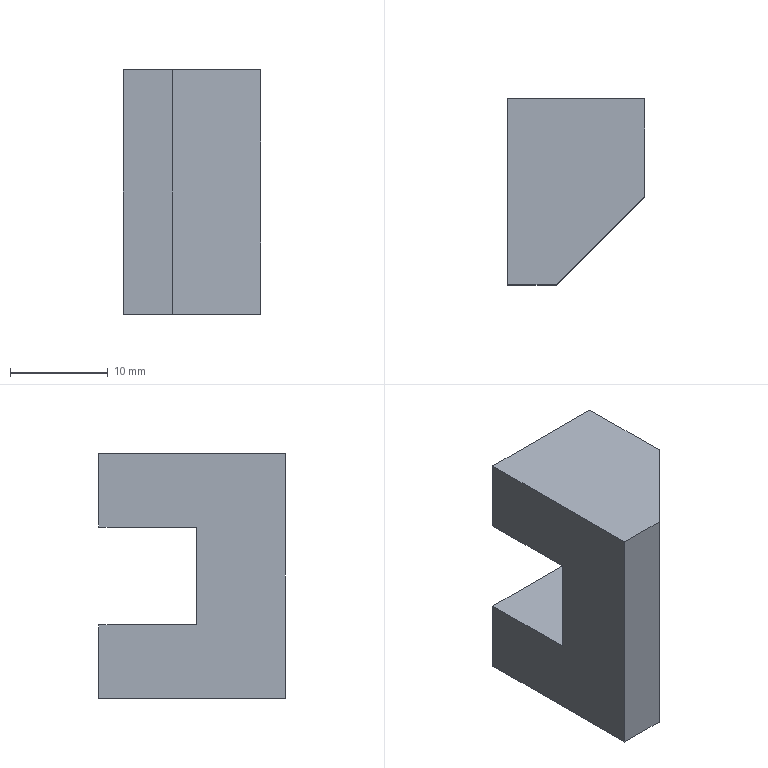Component | NX | CON_ROD4 | 1 solid | 12 faces | box 14 x 19 x 25 mm | volume 4238 mm3 | plane 12
STEP:
#1=CARTESIAN_POINT('',(0.,0.,0.));
#2=DIRECTION('',(0.,0.,1.));
#3=DIRECTION('',(1.,0.,0.));
#4=AXIS2_PLACEMENT_3D('',#1,#2,#3);
#5=CARTESIAN_POINT('',(101.5,69.,38.5));
#6=VERTEX_POINT('',#5);
#7=CARTESIAN_POINT('',(101.5,59.,38.5));
#8=VERTEX_POINT('',#7);
#9=CARTESIAN_POINT('',(101.5,69.,38.5));
#10=DIRECTION('',(0.,-1.,-0.));
#11=VECTOR('',#10,1.);
#12=LINE('',#9,#11);
#13=CARTESIAN_POINT('',(101.5,69.,26.));
#14=DIRECTION('',(1.,0.,0.));
#15=DIRECTION('',(0.,1.,0.));
#16=AXIS2_PLACEMENT_3D('',#13,#14,#15);
#17=PLANE('',#16);
#18=CARTESIAN_POINT('',(0.,12.5));
#19=DIRECTION('',(-1.,-0.));
#20=VECTOR('',#19,1.);
#21=LINE('',#18,#20);
#22=(GEOMETRIC_REPRESENTATION_CONTEXT(2)PARAMETRIC_REPRESENTATION_CONTEXT()REPRESENTATION_CONTEXT('',''));
#23=DEFINITIONAL_REPRESENTATION('',(#21),#22);
#24=PCURVE('',#17,#23);
#25=CARTESIAN_POINT('',(101.5,69.,38.5));
#26=DIRECTION('',(0.,0.,-1.));
#27=DIRECTION('',(0.,1.,0.));
#28=AXIS2_PLACEMENT_3D('',#25,#26,#27);
#29=PLANE('',#28);
#30=CARTESIAN_POINT('',(0.,0.));
#31=DIRECTION('',(-1.,0.));
#32=VECTOR('',#31,1.);
#33=LINE('',#30,#32);
#34=(GEOMETRIC_REPRESENTATION_CONTEXT(2)PARAMETRIC_REPRESENTATION_CONTEXT()REPRESENTATION_CONTEXT('',''));
#35=DEFINITIONAL_REPRESENTATION('',(#33),#34);
#36=PCURVE('',#29,#35);
#37=SURFACE_CURVE('',#12,(#24,#36),.PCURVE_S1.);
#38=EDGE_CURVE('',#6,#8,#37,.T.);
#39=ORIENTED_EDGE('',*,*,#38,.T.);
#40=CARTESIAN_POINT('',(101.5,59.,31.));
#41=VERTEX_POINT('',#40);
#42=CARTESIAN_POINT('',(101.5,59.,13.5));
#43=DIRECTION('',(0.,0.,-1.));
#44=VECTOR('',#43,1.);
#45=LINE('',#42,#44);
#46=CARTESIAN_POINT('',(-10.,-12.5));
#47=DIRECTION('',(0.,-1.));
#48=VECTOR('',#47,1.);
#49=LINE('',#46,#48);
#50=(GEOMETRIC_REPRESENTATION_CONTEXT(2)PARAMETRIC_REPRESENTATION_CONTEXT()REPRESENTATION_CONTEXT('',''));
#51=DEFINITIONAL_REPRESENTATION('',(#49),#50);
#52=PCURVE('',#17,#51);
#53=CARTESIAN_POINT('',(101.5,59.,26.));
#54=DIRECTION('',(0.7071,-0.7071,0.));
#55=DIRECTION('',(0.,0.,1.));
#56=AXIS2_PLACEMENT_3D('',#53,#54,#55);
#57=PLANE('',#56);
#58=CARTESIAN_POINT('',(-12.5,0.));
#59=DIRECTION('',(-1.,0.));
#60=VECTOR('',#59,1.);
#61=LINE('',#58,#60);
#62=(GEOMETRIC_REPRESENTATION_CONTEXT(2)PARAMETRIC_REPRESENTATION_CONTEXT()REPRESENTATION_CONTEXT('',''));
#63=DEFINITIONAL_REPRESENTATION('',(#61),#62);
#64=PCURVE('',#57,#63);
#65=SURFACE_CURVE('',#45,(#52,#64),.PCURVE_S1.);
#66=EDGE_CURVE('',#8,#41,#65,.T.);
#67=ORIENTED_EDGE('',*,*,#66,.T.);
#68=CARTESIAN_POINT('',(101.5,69.,31.));
#69=VERTEX_POINT('',#68);
#70=CARTESIAN_POINT('',(101.5,59.,31.));
#71=DIRECTION('',(0.,1.,0.));
#72=VECTOR('',#71,1.);
#73=LINE('',#70,#72);
#74=CARTESIAN_POINT('',(-10.,5.));
#75=DIRECTION('',(1.,0.));
#76=VECTOR('',#75,1.);
#77=LINE('',#74,#76);
#78=(GEOMETRIC_REPRESENTATION_CONTEXT(2)PARAMETRIC_REPRESENTATION_CONTEXT()REPRESENTATION_CONTEXT('',''));
#79=DEFINITIONAL_REPRESENTATION('',(#77),#78);
#80=PCURVE('',#17,#79);
#81=CARTESIAN_POINT('',(101.5,59.,31.));
#82=DIRECTION('',(0.,-0.,1.));
#83=DIRECTION('',(0.,-1.,-0.));
#84=AXIS2_PLACEMENT_3D('',#81,#82,#83);
#85=PLANE('',#84);
#86=CARTESIAN_POINT('',(0.,0.));
#87=DIRECTION('',(-1.,0.));
#88=VECTOR('',#87,1.);
#89=LINE('',#86,#88);
#90=(GEOMETRIC_REPRESENTATION_CONTEXT(2)PARAMETRIC_REPRESENTATION_CONTEXT()REPRESENTATION_CONTEXT('',''));
#91=DEFINITIONAL_REPRESENTATION('',(#89),#90);
#92=PCURVE('',#85,#91);
#93=SURFACE_CURVE('',#73,(#80,#92),.PCURVE_S1.);
#94=EDGE_CURVE('',#41,#69,#93,.T.);
#95=ORIENTED_EDGE('',*,*,#94,.T.);
#96=CARTESIAN_POINT('',(101.5,69.,31.));
#97=DIRECTION('',(0.,0.,1.));
#98=VECTOR('',#97,1.);
#99=LINE('',#96,#98);
#100=CARTESIAN_POINT('',(0.,5.));
#101=DIRECTION('',(0.,1.));
#102=VECTOR('',#101,1.);
#103=LINE('',#100,#102);
#104=(GEOMETRIC_REPRESENTATION_CONTEXT(2)PARAMETRIC_REPRESENTATION_CONTEXT()REPRESENTATION_CONTEXT('',''));
#105=DEFINITIONAL_REPRESENTATION('',(#103),#104);
#106=PCURVE('',#17,#105);
#107=CARTESIAN_POINT('',(101.5,69.,31.));
#108=DIRECTION('',(0.,-1.,0.));
#109=DIRECTION('',(1.,0.,0.));
#110=AXIS2_PLACEMENT_3D('',#107,#108,#109);
#111=PLANE('',#110);
#112=CARTESIAN_POINT('',(0.,0.));
#113=DIRECTION('',(0.,1.));
#114=VECTOR('',#113,1.);
#115=LINE('',#112,#114);
#116=(GEOMETRIC_REPRESENTATION_CONTEXT(2)PARAMETRIC_REPRESENTATION_CONTEXT()REPRESENTATION_CONTEXT('',''));
#117=DEFINITIONAL_REPRESENTATION('',(#115),#116);
#118=PCURVE('',#111,#117);
#119=SURFACE_CURVE('',#99,(#106,#118),.PCURVE_S1.);
#120=EDGE_CURVE('',#69,#6,#119,.T.);
#121=ORIENTED_EDGE('',*,*,#120,.T.);
#122=EDGE_LOOP('',(#39,#67,#95,#121));
#123=FACE_BOUND('',#122,.T.);
#124=ADVANCED_FACE('',(#123),#17,.T.);
#125=CARTESIAN_POINT('',(101.5,59.,13.5));
#126=VERTEX_POINT('',#125);
#127=CARTESIAN_POINT('',(101.5,69.,13.5));
#128=VERTEX_POINT('',#127);
#129=CARTESIAN_POINT('',(101.5,50.,13.5));
#130=DIRECTION('',(0.,1.,0.));
#131=VECTOR('',#130,1.);
#132=LINE('',#129,#131);
#133=CARTESIAN_POINT('',(101.5,50.,13.5));
#134=DIRECTION('',(0.,-0.,1.));
#135=DIRECTION('',(0.,-1.,-0.));
#136=AXIS2_PLACEMENT_3D('',#133,#134,#135);
#137=PLANE('',#136);
#138=CARTESIAN_POINT('',(0.,0.));
#139=DIRECTION('',(-1.,0.));
#140=VECTOR('',#139,1.);
#141=LINE('',#138,#140);
#142=(GEOMETRIC_REPRESENTATION_CONTEXT(2)PARAMETRIC_REPRESENTATION_CONTEXT()REPRESENTATION_CONTEXT('',''));
#143=DEFINITIONAL_REPRESENTATION('',(#141),#142);
#144=PCURVE('',#137,#143);
#145=CARTESIAN_POINT('',(101.5,69.,26.));
#146=DIRECTION('',(1.,0.,0.));
#147=DIRECTION('',(0.,1.,0.));
#148=AXIS2_PLACEMENT_3D('',#145,#146,#147);
#149=PLANE('',#148);
#150=CARTESIAN_POINT('',(-19.,-12.5));
#151=DIRECTION('',(1.,0.));
#152=VECTOR('',#151,1.);
#153=LINE('',#150,#152);
#154=(GEOMETRIC_REPRESENTATION_CONTEXT(2)PARAMETRIC_REPRESENTATION_CONTEXT()REPRESENTATION_CONTEXT('',''));
#155=DEFINITIONAL_REPRESENTATION('',(#153),#154);
#156=PCURVE('',#149,#155);
#157=SURFACE_CURVE('',#132,(#144,#156),.PCURVE_S1.);
#158=EDGE_CURVE('',#126,#128,#157,.T.);
#159=ORIENTED_EDGE('',*,*,#158,.F.);
#160=CARTESIAN_POINT('',(92.5,50.,13.5));
#161=VERTEX_POINT('',#160);
#162=CARTESIAN_POINT('',(101.5,59.,13.5));
#163=DIRECTION('',(-0.7071,-0.7071,-0.));
#164=VECTOR('',#163,1.);
#165=LINE('',#162,#164);
#166=CARTESIAN_POINT('',(-9.,0.));
#167=DIRECTION('',(0.7071,-0.7071));
#168=VECTOR('',#167,1.);
#169=LINE('',#166,#168);
#170=(GEOMETRIC_REPRESENTATION_CONTEXT(2)PARAMETRIC_REPRESENTATION_CONTEXT()REPRESENTATION_CONTEXT('',''));
#171=DEFINITIONAL_REPRESENTATION('',(#169),#170);
#172=PCURVE('',#137,#171);
#173=CARTESIAN_POINT('',(-12.5,0.));
#174=DIRECTION('',(-0.,1.));
#175=VECTOR('',#174,1.);
#176=LINE('',#173,#175);
#177=(GEOMETRIC_REPRESENTATION_CONTEXT(2)PARAMETRIC_REPRESENTATION_CONTEXT()REPRESENTATION_CONTEXT('',''));
#178=DEFINITIONAL_REPRESENTATION('',(#176),#177);
#179=PCURVE('',#57,#178);
#180=SURFACE_CURVE('',#165,(#172,#179),.PCURVE_S1.);
#181=EDGE_CURVE('',#126,#161,#180,.T.);
#182=ORIENTED_EDGE('',*,*,#181,.T.);
#183=CARTESIAN_POINT('',(87.5,50.,13.5));
#184=VERTEX_POINT('',#183);
#185=CARTESIAN_POINT('',(101.5,50.,13.5));
#186=DIRECTION('',(-1.,0.,0.));
#187=VECTOR('',#186,1.);
#188=LINE('',#185,#187);
#189=CARTESIAN_POINT('',(0.,0.));
#190=DIRECTION('',(0.,-1.));
#191=VECTOR('',#190,1.);
#192=LINE('',#189,#191);
#193=(GEOMETRIC_REPRESENTATION_CONTEXT(2)PARAMETRIC_REPRESENTATION_CONTEXT()REPRESENTATION_CONTEXT('',''));
#194=DEFINITIONAL_REPRESENTATION('',(#192),#193);
#195=PCURVE('',#137,#194);
#196=CARTESIAN_POINT('',(101.5,50.,38.5));
#197=DIRECTION('',(0.,1.,0.));
#198=DIRECTION('',(-1.,0.,0.));
#199=AXIS2_PLACEMENT_3D('',#196,#197,#198);
#200=PLANE('',#199);
#201=CARTESIAN_POINT('',(0.,-25.));
#202=DIRECTION('',(1.,0.));
#203=VECTOR('',#202,1.);
#204=LINE('',#201,#203);
#205=(GEOMETRIC_REPRESENTATION_CONTEXT(2)PARAMETRIC_REPRESENTATION_CONTEXT()REPRESENTATION_CONTEXT('',''));
#206=DEFINITIONAL_REPRESENTATION('',(#204),#205);
#207=PCURVE('',#200,#206);
#208=SURFACE_CURVE('',#188,(#195,#207),.PCURVE_S1.);
#209=EDGE_CURVE('',#161,#184,#208,.T.);
#210=ORIENTED_EDGE('',*,*,#209,.T.);
#211=CARTESIAN_POINT('',(87.5,69.,13.5));
#212=VERTEX_POINT('',#211);
#213=CARTESIAN_POINT('',(87.5,50.,13.5));
#214=DIRECTION('',(0.,1.,0.));
#215=VECTOR('',#214,1.);
#216=LINE('',#213,#215);
#217=CARTESIAN_POINT('',(0.,-14.));
#218=DIRECTION('',(-1.,0.));
#219=VECTOR('',#218,1.);
#220=LINE('',#217,#219);
#221=(GEOMETRIC_REPRESENTATION_CONTEXT(2)PARAMETRIC_REPRESENTATION_CONTEXT()REPRESENTATION_CONTEXT('',''));
#222=DEFINITIONAL_REPRESENTATION('',(#220),#221);
#223=PCURVE('',#137,#222);
#224=CARTESIAN_POINT('',(87.5,69.,26.));
#225=DIRECTION('',(1.,0.,0.));
#226=DIRECTION('',(0.,1.,0.));
#227=AXIS2_PLACEMENT_3D('',#224,#225,#226);
#228=PLANE('',#227);
#229=CARTESIAN_POINT('',(-19.,-12.5));
#230=DIRECTION('',(1.,0.));
#231=VECTOR('',#230,1.);
#232=LINE('',#229,#231);
#233=(GEOMETRIC_REPRESENTATION_CONTEXT(2)PARAMETRIC_REPRESENTATION_CONTEXT()REPRESENTATION_CONTEXT('',''));
#234=DEFINITIONAL_REPRESENTATION('',(#232),#233);
#235=PCURVE('',#228,#234);
#236=SURFACE_CURVE('',#216,(#223,#235),.PCURVE_S1.);
#237=EDGE_CURVE('',#184,#212,#236,.T.);
#238=ORIENTED_EDGE('',*,*,#237,.T.);
#239=CARTESIAN_POINT('',(101.5,69.,13.5));
#240=DIRECTION('',(-1.,0.,0.));
#241=VECTOR('',#240,1.);
#242=LINE('',#239,#241);
#243=CARTESIAN_POINT('',(-19.,0.));
#244=DIRECTION('',(0.,-1.));
#245=VECTOR('',#244,1.);
#246=LINE('',#243,#245);
#247=(GEOMETRIC_REPRESENTATION_CONTEXT(2)PARAMETRIC_REPRESENTATION_CONTEXT()REPRESENTATION_CONTEXT('',''));
#248=DEFINITIONAL_REPRESENTATION('',(#246),#247);
#249=PCURVE('',#137,#248);
#250=CARTESIAN_POINT('',(101.5,69.,13.5));
#251=DIRECTION('',(0.,-1.,0.));
#252=DIRECTION('',(1.,0.,0.));
#253=AXIS2_PLACEMENT_3D('',#250,#251,#252);
#254=PLANE('',#253);
#255=CARTESIAN_POINT('',(0.,0.));
#256=DIRECTION('',(-1.,0.));
#257=VECTOR('',#256,1.);
#258=LINE('',#255,#257);
#259=(GEOMETRIC_REPRESENTATION_CONTEXT(2)PARAMETRIC_REPRESENTATION_CONTEXT()REPRESENTATION_CONTEXT('',''));
#260=DEFINITIONAL_REPRESENTATION('',(#258),#259);
#261=PCURVE('',#254,#260);
#262=SURFACE_CURVE('',#242,(#249,#261),.PCURVE_S1.);
#263=EDGE_CURVE('',#128,#212,#262,.T.);
#264=ORIENTED_EDGE('',*,*,#263,.F.);
#265=EDGE_LOOP('',(#159,#182,#210,#238,#264));
#266=FACE_BOUND('',#265,.T.);
#267=ADVANCED_FACE('',(#266),#137,.F.);
#268=CARTESIAN_POINT('',(87.5,69.,21.));
#269=VERTEX_POINT('',#268);
#270=CARTESIAN_POINT('',(87.5,69.,13.5));
#271=DIRECTION('',(0.,0.,1.));
#272=VECTOR('',#271,1.);
#273=LINE('',#270,#272);
#274=CARTESIAN_POINT('',(-14.,0.));
#275=DIRECTION('',(0.,1.));
#276=VECTOR('',#275,1.);
#277=LINE('',#274,#276);
#278=(GEOMETRIC_REPRESENTATION_CONTEXT(2)PARAMETRIC_REPRESENTATION_CONTEXT()REPRESENTATION_CONTEXT('',''));
#279=DEFINITIONAL_REPRESENTATION('',(#277),#278);
#280=PCURVE('',#254,#279);
#281=CARTESIAN_POINT('',(0.,-12.5));
#282=DIRECTION('',(0.,1.));
#283=VECTOR('',#282,1.);
#284=LINE('',#281,#283);
#285=(GEOMETRIC_REPRESENTATION_CONTEXT(2)PARAMETRIC_REPRESENTATION_CONTEXT()REPRESENTATION_CONTEXT('',''));
#286=DEFINITIONAL_REPRESENTATION('',(#284),#285);
#287=PCURVE('',#228,#286);
#288=SURFACE_CURVE('',#273,(#280,#287),.PCURVE_S1.);
#289=EDGE_CURVE('',#212,#269,#288,.T.);
#290=ORIENTED_EDGE('',*,*,#289,.T.);
#291=CARTESIAN_POINT('',(101.5,69.,21.));
#292=VERTEX_POINT('',#291);
#293=CARTESIAN_POINT('',(101.5,69.,21.));
#294=DIRECTION('',(-1.,0.,0.));
#295=VECTOR('',#294,1.);
#296=LINE('',#293,#295);
#297=CARTESIAN_POINT('',(0.,7.5));
#298=DIRECTION('',(-1.,0.));
#299=VECTOR('',#298,1.);
#300=LINE('',#297,#299);
#301=(GEOMETRIC_REPRESENTATION_CONTEXT(2)PARAMETRIC_REPRESENTATION_CONTEXT()REPRESENTATION_CONTEXT('',''));
#302=DEFINITIONAL_REPRESENTATION('',(#300),#301);
#303=PCURVE('',#254,#302);
#304=CARTESIAN_POINT('',(101.5,69.,21.));
#305=DIRECTION('',(0.,0.,-1.));
#306=DIRECTION('',(0.,1.,0.));
#307=AXIS2_PLACEMENT_3D('',#304,#305,#306);
#308=PLANE('',#307);
#309=CARTESIAN_POINT('',(0.,0.));
#310=DIRECTION('',(0.,-1.));
#311=VECTOR('',#310,1.);
#312=LINE('',#309,#311);
#313=(GEOMETRIC_REPRESENTATION_CONTEXT(2)PARAMETRIC_REPRESENTATION_CONTEXT()REPRESENTATION_CONTEXT('',''));
#314=DEFINITIONAL_REPRESENTATION('',(#312),#313);
#315=PCURVE('',#308,#314);
#316=SURFACE_CURVE('',#296,(#303,#315),.PCURVE_S1.);
#317=EDGE_CURVE('',#292,#269,#316,.T.);
#318=ORIENTED_EDGE('',*,*,#317,.F.);
#319=CARTESIAN_POINT('',(101.5,69.,13.5));
#320=DIRECTION('',(0.,0.,1.));
#321=VECTOR('',#320,1.);
#322=LINE('',#319,#321);
#323=CARTESIAN_POINT('',(0.,0.));
#324=DIRECTION('',(0.,1.));
#325=VECTOR('',#324,1.);
#326=LINE('',#323,#325);
#327=(GEOMETRIC_REPRESENTATION_CONTEXT(2)PARAMETRIC_REPRESENTATION_CONTEXT()REPRESENTATION_CONTEXT('',''));
#328=DEFINITIONAL_REPRESENTATION('',(#326),#327);
#329=PCURVE('',#254,#328);
#330=CARTESIAN_POINT('',(0.,-12.5));
#331=DIRECTION('',(0.,1.));
#332=VECTOR('',#331,1.);
#333=LINE('',#330,#332);
#334=(GEOMETRIC_REPRESENTATION_CONTEXT(2)PARAMETRIC_REPRESENTATION_CONTEXT()REPRESENTATION_CONTEXT('',''));
#335=DEFINITIONAL_REPRESENTATION('',(#333),#334);
#336=PCURVE('',#149,#335);
#337=SURFACE_CURVE('',#322,(#329,#336),.PCURVE_S1.);
#338=EDGE_CURVE('',#128,#292,#337,.T.);
#339=ORIENTED_EDGE('',*,*,#338,.F.);
#340=ORIENTED_EDGE('',*,*,#263,.T.);
#341=EDGE_LOOP('',(#290,#318,#339,#340));
#342=FACE_BOUND('',#341,.T.);
#343=ADVANCED_FACE('',(#342),#254,.F.);
#344=CARTESIAN_POINT('',(87.5,59.,21.));
#345=VERTEX_POINT('',#344);
#346=CARTESIAN_POINT('',(87.5,69.,21.));
#347=DIRECTION('',(0.,-1.,0.));
#348=VECTOR('',#347,1.);
#349=LINE('',#346,#348);
#350=CARTESIAN_POINT('',(0.,-14.));
#351=DIRECTION('',(-1.,0.));
#352=VECTOR('',#351,1.);
#353=LINE('',#350,#352);
#354=(GEOMETRIC_REPRESENTATION_CONTEXT(2)PARAMETRIC_REPRESENTATION_CONTEXT()REPRESENTATION_CONTEXT('',''));
#355=DEFINITIONAL_REPRESENTATION('',(#353),#354);
#356=PCURVE('',#308,#355);
#357=CARTESIAN_POINT('',(0.,-5.));
#358=DIRECTION('',(-1.,0.));
#359=VECTOR('',#358,1.);
#360=LINE('',#357,#359);
#361=(GEOMETRIC_REPRESENTATION_CONTEXT(2)PARAMETRIC_REPRESENTATION_CONTEXT()REPRESENTATION_CONTEXT('',''));
#362=DEFINITIONAL_REPRESENTATION('',(#360),#361);
#363=PCURVE('',#228,#362);
#364=SURFACE_CURVE('',#349,(#356,#363),.PCURVE_S1.);
#365=EDGE_CURVE('',#269,#345,#364,.T.);
#366=ORIENTED_EDGE('',*,*,#365,.T.);
#367=CARTESIAN_POINT('',(101.5,59.,21.));
#368=VERTEX_POINT('',#367);
#369=CARTESIAN_POINT('',(101.5,59.,21.));
#370=DIRECTION('',(-1.,0.,0.));
#371=VECTOR('',#370,1.);
#372=LINE('',#369,#371);
#373=CARTESIAN_POINT('',(-10.,0.));
#374=DIRECTION('',(0.,-1.));
#375=VECTOR('',#374,1.);
#376=LINE('',#373,#375);
#377=(GEOMETRIC_REPRESENTATION_CONTEXT(2)PARAMETRIC_REPRESENTATION_CONTEXT()REPRESENTATION_CONTEXT('',''));
#378=DEFINITIONAL_REPRESENTATION('',(#376),#377);
#379=PCURVE('',#308,#378);
#380=CARTESIAN_POINT('',(101.5,59.,21.));
#381=DIRECTION('',(0.,-1.,-0.));
#382=DIRECTION('',(0.,0.,-1.));
#383=AXIS2_PLACEMENT_3D('',#380,#381,#382);
#384=PLANE('',#383);
#385=CARTESIAN_POINT('',(0.,0.));
#386=DIRECTION('',(0.,-1.));
#387=VECTOR('',#386,1.);
#388=LINE('',#385,#387);
#389=(GEOMETRIC_REPRESENTATION_CONTEXT(2)PARAMETRIC_REPRESENTATION_CONTEXT()REPRESENTATION_CONTEXT('',''));
#390=DEFINITIONAL_REPRESENTATION('',(#388),#389);
#391=PCURVE('',#384,#390);
#392=SURFACE_CURVE('',#372,(#379,#391),.PCURVE_S1.);
#393=EDGE_CURVE('',#368,#345,#392,.T.);
#394=ORIENTED_EDGE('',*,*,#393,.F.);
#395=CARTESIAN_POINT('',(101.5,69.,21.));
#396=DIRECTION('',(0.,-1.,0.));
#397=VECTOR('',#396,1.);
#398=LINE('',#395,#397);
#399=CARTESIAN_POINT('',(0.,0.));
#400=DIRECTION('',(-1.,0.));
#401=VECTOR('',#400,1.);
#402=LINE('',#399,#401);
#403=(GEOMETRIC_REPRESENTATION_CONTEXT(2)PARAMETRIC_REPRESENTATION_CONTEXT()REPRESENTATION_CONTEXT('',''));
#404=DEFINITIONAL_REPRESENTATION('',(#402),#403);
#405=PCURVE('',#308,#404);
#406=CARTESIAN_POINT('',(0.,-5.));
#407=DIRECTION('',(-1.,0.));
#408=VECTOR('',#407,1.);
#409=LINE('',#406,#408);
#410=(GEOMETRIC_REPRESENTATION_CONTEXT(2)PARAMETRIC_REPRESENTATION_CONTEXT()REPRESENTATION_CONTEXT('',''));
#411=DEFINITIONAL_REPRESENTATION('',(#409),#410);
#412=PCURVE('',#149,#411);
#413=SURFACE_CURVE('',#398,(#405,#412),.PCURVE_S1.);
#414=EDGE_CURVE('',#292,#368,#413,.T.);
#415=ORIENTED_EDGE('',*,*,#414,.F.);
#416=ORIENTED_EDGE('',*,*,#317,.T.);
#417=EDGE_LOOP('',(#366,#394,#415,#416));
#418=FACE_BOUND('',#417,.T.);
#419=ADVANCED_FACE('',(#418),#308,.F.);
#420=CARTESIAN_POINT('',(87.5,59.,31.));
#421=VERTEX_POINT('',#420);
#422=CARTESIAN_POINT('',(87.5,59.,21.));
#423=DIRECTION('',(0.,-0.,1.));
#424=VECTOR('',#423,1.);
#425=LINE('',#422,#424);
#426=CARTESIAN_POINT('',(0.,-14.));
#427=DIRECTION('',(-1.,0.));
#428=VECTOR('',#427,1.);
#429=LINE('',#426,#428);
#430=(GEOMETRIC_REPRESENTATION_CONTEXT(2)PARAMETRIC_REPRESENTATION_CONTEXT()REPRESENTATION_CONTEXT('',''));
#431=DEFINITIONAL_REPRESENTATION('',(#429),#430);
#432=PCURVE('',#384,#431);
#433=CARTESIAN_POINT('',(-10.,-5.));
#434=DIRECTION('',(-0.,1.));
#435=VECTOR('',#434,1.);
#436=LINE('',#433,#435);
#437=(GEOMETRIC_REPRESENTATION_CONTEXT(2)PARAMETRIC_REPRESENTATION_CONTEXT()REPRESENTATION_CONTEXT('',''));
#438=DEFINITIONAL_REPRESENTATION('',(#436),#437);
#439=PCURVE('',#228,#438);
#440=SURFACE_CURVE('',#425,(#432,#439),.PCURVE_S1.);
#441=EDGE_CURVE('',#345,#421,#440,.T.);
#442=ORIENTED_EDGE('',*,*,#441,.T.);
#443=CARTESIAN_POINT('',(101.5,59.,31.));
#444=DIRECTION('',(-1.,0.,0.));
#445=VECTOR('',#444,1.);
#446=LINE('',#443,#445);
#447=CARTESIAN_POINT('',(-10.,0.));
#448=DIRECTION('',(0.,-1.));
#449=VECTOR('',#448,1.);
#450=LINE('',#447,#449);
#451=(GEOMETRIC_REPRESENTATION_CONTEXT(2)PARAMETRIC_REPRESENTATION_CONTEXT()REPRESENTATION_CONTEXT('',''));
#452=DEFINITIONAL_REPRESENTATION('',(#450),#451);
#453=PCURVE('',#384,#452);
#454=CARTESIAN_POINT('',(0.,0.));
#455=DIRECTION('',(0.,-1.));
#456=VECTOR('',#455,1.);
#457=LINE('',#454,#456);
#458=(GEOMETRIC_REPRESENTATION_CONTEXT(2)PARAMETRIC_REPRESENTATION_CONTEXT()REPRESENTATION_CONTEXT('',''));
#459=DEFINITIONAL_REPRESENTATION('',(#457),#458);
#460=PCURVE('',#85,#459);
#461=SURFACE_CURVE('',#446,(#453,#460),.PCURVE_S1.);
#462=EDGE_CURVE('',#41,#421,#461,.T.);
#463=ORIENTED_EDGE('',*,*,#462,.F.);
#464=CARTESIAN_POINT('',(101.5,59.,21.));
#465=DIRECTION('',(0.,-0.,1.));
#466=VECTOR('',#465,1.);
#467=LINE('',#464,#466);
#468=CARTESIAN_POINT('',(0.,0.));
#469=DIRECTION('',(-1.,0.));
#470=VECTOR('',#469,1.);
#471=LINE('',#468,#470);
#472=(GEOMETRIC_REPRESENTATION_CONTEXT(2)PARAMETRIC_REPRESENTATION_CONTEXT()REPRESENTATION_CONTEXT('',''));
#473=DEFINITIONAL_REPRESENTATION('',(#471),#472);
#474=PCURVE('',#384,#473);
#475=CARTESIAN_POINT('',(-5.,0.));
#476=DIRECTION('',(1.,0.));
#477=VECTOR('',#476,1.);
#478=LINE('',#475,#477);
#479=(GEOMETRIC_REPRESENTATION_CONTEXT(2)PARAMETRIC_REPRESENTATION_CONTEXT()REPRESENTATION_CONTEXT('',''));
#480=DEFINITIONAL_REPRESENTATION('',(#478),#479);
#481=PCURVE('',#57,#480);
#482=SURFACE_CURVE('',#467,(#474,#481),.PCURVE_S1.);
#483=EDGE_CURVE('',#368,#41,#482,.T.);
#484=ORIENTED_EDGE('',*,*,#483,.F.);
#485=ORIENTED_EDGE('',*,*,#393,.T.);
#486=EDGE_LOOP('',(#442,#463,#484,#485));
#487=FACE_BOUND('',#486,.T.);
#488=ADVANCED_FACE('',(#487),#384,.F.);
#489=CARTESIAN_POINT('',(87.5,69.,31.));
#490=VERTEX_POINT('',#489);
#491=CARTESIAN_POINT('',(87.5,59.,31.));
#492=DIRECTION('',(0.,1.,0.));
#493=VECTOR('',#492,1.);
#494=LINE('',#491,#493);
#495=CARTESIAN_POINT('',(0.,-14.));
#496=DIRECTION('',(-1.,0.));
#497=VECTOR('',#496,1.);
#498=LINE('',#495,#497);
#499=(GEOMETRIC_REPRESENTATION_CONTEXT(2)PARAMETRIC_REPRESENTATION_CONTEXT()REPRESENTATION_CONTEXT('',''));
#500=DEFINITIONAL_REPRESENTATION('',(#498),#499);
#501=PCURVE('',#85,#500);
#502=CARTESIAN_POINT('',(-10.,5.));
#503=DIRECTION('',(1.,0.));
#504=VECTOR('',#503,1.);
#505=LINE('',#502,#504);
#506=(GEOMETRIC_REPRESENTATION_CONTEXT(2)PARAMETRIC_REPRESENTATION_CONTEXT()REPRESENTATION_CONTEXT('',''));
#507=DEFINITIONAL_REPRESENTATION('',(#505),#506);
#508=PCURVE('',#228,#507);
#509=SURFACE_CURVE('',#494,(#501,#508),.PCURVE_S1.);
#510=EDGE_CURVE('',#421,#490,#509,.T.);
#511=ORIENTED_EDGE('',*,*,#510,.T.);
#512=CARTESIAN_POINT('',(101.5,69.,31.));
#513=DIRECTION('',(-1.,0.,0.));
#514=VECTOR('',#513,1.);
#515=LINE('',#512,#514);
#516=CARTESIAN_POINT('',(-10.,0.));
#517=DIRECTION('',(0.,-1.));
#518=VECTOR('',#517,1.);
#519=LINE('',#516,#518);
#520=(GEOMETRIC_REPRESENTATION_CONTEXT(2)PARAMETRIC_REPRESENTATION_CONTEXT()REPRESENTATION_CONTEXT('',''));
#521=DEFINITIONAL_REPRESENTATION('',(#519),#520);
#522=PCURVE('',#85,#521);
#523=CARTESIAN_POINT('',(0.,0.));
#524=DIRECTION('',(-1.,0.));
#525=VECTOR('',#524,1.);
#526=LINE('',#523,#525);
#527=(GEOMETRIC_REPRESENTATION_CONTEXT(2)PARAMETRIC_REPRESENTATION_CONTEXT()REPRESENTATION_CONTEXT('',''));
#528=DEFINITIONAL_REPRESENTATION('',(#526),#527);
#529=PCURVE('',#111,#528);
#530=SURFACE_CURVE('',#515,(#522,#529),.PCURVE_S1.);
#531=EDGE_CURVE('',#69,#490,#530,.T.);
#532=ORIENTED_EDGE('',*,*,#531,.F.);
#533=ORIENTED_EDGE('',*,*,#94,.F.);
#534=ORIENTED_EDGE('',*,*,#462,.T.);
#535=EDGE_LOOP('',(#511,#532,#533,#534));
#536=FACE_BOUND('',#535,.T.);
#537=ADVANCED_FACE('',(#536),#85,.F.);
#538=CARTESIAN_POINT('',(87.5,69.,38.5));
#539=VERTEX_POINT('',#538);
#540=CARTESIAN_POINT('',(87.5,69.,31.));
#541=DIRECTION('',(0.,0.,1.));
#542=VECTOR('',#541,1.);
#543=LINE('',#540,#542);
#544=CARTESIAN_POINT('',(-14.,0.));
#545=DIRECTION('',(0.,1.));
#546=VECTOR('',#545,1.);
#547=LINE('',#544,#546);
#548=(GEOMETRIC_REPRESENTATION_CONTEXT(2)PARAMETRIC_REPRESENTATION_CONTEXT()REPRESENTATION_CONTEXT('',''));
#549=DEFINITIONAL_REPRESENTATION('',(#547),#548);
#550=PCURVE('',#111,#549);
#551=CARTESIAN_POINT('',(0.,5.));
#552=DIRECTION('',(0.,1.));
#553=VECTOR('',#552,1.);
#554=LINE('',#551,#553);
#555=(GEOMETRIC_REPRESENTATION_CONTEXT(2)PARAMETRIC_REPRESENTATION_CONTEXT()REPRESENTATION_CONTEXT('',''));
#556=DEFINITIONAL_REPRESENTATION('',(#554),#555);
#557=PCURVE('',#228,#556);
#558=SURFACE_CURVE('',#543,(#550,#557),.PCURVE_S1.);
#559=EDGE_CURVE('',#490,#539,#558,.T.);
#560=ORIENTED_EDGE('',*,*,#559,.T.);
#561=CARTESIAN_POINT('',(101.5,69.,38.5));
#562=DIRECTION('',(-1.,0.,0.));
#563=VECTOR('',#562,1.);
#564=LINE('',#561,#563);
#565=CARTESIAN_POINT('',(0.,7.5));
#566=DIRECTION('',(-1.,0.));
#567=VECTOR('',#566,1.);
#568=LINE('',#565,#567);
#569=(GEOMETRIC_REPRESENTATION_CONTEXT(2)PARAMETRIC_REPRESENTATION_CONTEXT()REPRESENTATION_CONTEXT('',''));
#570=DEFINITIONAL_REPRESENTATION('',(#568),#569);
#571=PCURVE('',#111,#570);
#572=CARTESIAN_POINT('',(0.,0.));
#573=DIRECTION('',(0.,-1.));
#574=VECTOR('',#573,1.);
#575=LINE('',#572,#574);
#576=(GEOMETRIC_REPRESENTATION_CONTEXT(2)PARAMETRIC_REPRESENTATION_CONTEXT()REPRESENTATION_CONTEXT('',''));
#577=DEFINITIONAL_REPRESENTATION('',(#575),#576);
#578=PCURVE('',#29,#577);
#579=SURFACE_CURVE('',#564,(#571,#578),.PCURVE_S1.);
#580=EDGE_CURVE('',#6,#539,#579,.T.);
#581=ORIENTED_EDGE('',*,*,#580,.F.);
#582=ORIENTED_EDGE('',*,*,#120,.F.);
#583=ORIENTED_EDGE('',*,*,#531,.T.);
#584=EDGE_LOOP('',(#560,#581,#582,#583));
#585=FACE_BOUND('',#584,.T.);
#586=ADVANCED_FACE('',(#585),#111,.F.);
#587=CARTESIAN_POINT('',(92.5,50.,38.5));
#588=VERTEX_POINT('',#587);
#589=CARTESIAN_POINT('',(87.5,50.,38.5));
#590=VERTEX_POINT('',#589);
#591=CARTESIAN_POINT('',(101.5,50.,38.5));
#592=DIRECTION('',(-1.,0.,0.));
#593=VECTOR('',#592,1.);
#594=LINE('',#591,#593);
#595=CARTESIAN_POINT('',(-19.,0.));
#596=DIRECTION('',(0.,-1.));
#597=VECTOR('',#596,1.);
#598=LINE('',#595,#597);
#599=(GEOMETRIC_REPRESENTATION_CONTEXT(2)PARAMETRIC_REPRESENTATION_CONTEXT()REPRESENTATION_CONTEXT('',''));
#600=DEFINITIONAL_REPRESENTATION('',(#598),#599);
#601=PCURVE('',#29,#600);
#602=CARTESIAN_POINT('',(0.,0.));
#603=DIRECTION('',(1.,0.));
#604=VECTOR('',#603,1.);
#605=LINE('',#602,#604);
#606=(GEOMETRIC_REPRESENTATION_CONTEXT(2)PARAMETRIC_REPRESENTATION_CONTEXT()REPRESENTATION_CONTEXT('',''));
#607=DEFINITIONAL_REPRESENTATION('',(#605),#606);
#608=PCURVE('',#200,#607);
#609=SURFACE_CURVE('',#594,(#601,#608),.PCURVE_S1.);
#610=EDGE_CURVE('',#588,#590,#609,.T.);
#611=ORIENTED_EDGE('',*,*,#610,.F.);
#612=CARTESIAN_POINT('',(101.5,59.,38.5));
#613=DIRECTION('',(0.7071,0.7071,0.));
#614=VECTOR('',#613,1.);
#615=LINE('',#612,#614);
#616=CARTESIAN_POINT('',(-10.,0.));
#617=DIRECTION('',(0.7071,0.7071));
#618=VECTOR('',#617,1.);
#619=LINE('',#616,#618);
#620=(GEOMETRIC_REPRESENTATION_CONTEXT(2)PARAMETRIC_REPRESENTATION_CONTEXT()REPRESENTATION_CONTEXT('',''));
#621=DEFINITIONAL_REPRESENTATION('',(#619),#620);
#622=PCURVE('',#29,#621);
#623=CARTESIAN_POINT('',(12.5,0.));
#624=DIRECTION('',(0.,-1.));
#625=VECTOR('',#624,1.);
#626=LINE('',#623,#625);
#627=(GEOMETRIC_REPRESENTATION_CONTEXT(2)PARAMETRIC_REPRESENTATION_CONTEXT()REPRESENTATION_CONTEXT('',''));
#628=DEFINITIONAL_REPRESENTATION('',(#626),#627);
#629=PCURVE('',#57,#628);
#630=SURFACE_CURVE('',#615,(#622,#629),.PCURVE_S1.);
#631=EDGE_CURVE('',#588,#8,#630,.T.);
#632=ORIENTED_EDGE('',*,*,#631,.T.);
#633=ORIENTED_EDGE('',*,*,#38,.F.);
#634=ORIENTED_EDGE('',*,*,#580,.T.);
#635=CARTESIAN_POINT('',(87.5,69.,38.5));
#636=DIRECTION('',(0.,-1.,-0.));
#637=VECTOR('',#636,1.);
#638=LINE('',#635,#637);
#639=CARTESIAN_POINT('',(0.,-14.));
#640=DIRECTION('',(-1.,0.));
#641=VECTOR('',#640,1.);
#642=LINE('',#639,#641);
#643=(GEOMETRIC_REPRESENTATION_CONTEXT(2)PARAMETRIC_REPRESENTATION_CONTEXT()REPRESENTATION_CONTEXT('',''));
#644=DEFINITIONAL_REPRESENTATION('',(#642),#643);
#645=PCURVE('',#29,#644);
#646=CARTESIAN_POINT('',(0.,12.5));
#647=DIRECTION('',(-1.,-0.));
#648=VECTOR('',#647,1.);
#649=LINE('',#646,#648);
#650=(GEOMETRIC_REPRESENTATION_CONTEXT(2)PARAMETRIC_REPRESENTATION_CONTEXT()REPRESENTATION_CONTEXT('',''));
#651=DEFINITIONAL_REPRESENTATION('',(#649),#650);
#652=PCURVE('',#228,#651);
#653=SURFACE_CURVE('',#638,(#645,#652),.PCURVE_S1.);
#654=EDGE_CURVE('',#539,#590,#653,.T.);
#655=ORIENTED_EDGE('',*,*,#654,.T.);
#656=EDGE_LOOP('',(#611,#632,#633,#634,#655));
#657=FACE_BOUND('',#656,.T.);
#658=ADVANCED_FACE('',(#657),#29,.F.);
#659=ORIENTED_EDGE('',*,*,#209,.F.);
#660=CARTESIAN_POINT('',(92.5,50.,38.5));
#661=DIRECTION('',(0.,0.,1.));
#662=VECTOR('',#661,1.);
#663=LINE('',#660,#662);
#664=CARTESIAN_POINT('',(9.,0.));
#665=DIRECTION('',(0.,1.));
#666=VECTOR('',#665,1.);
#667=LINE('',#664,#666);
#668=(GEOMETRIC_REPRESENTATION_CONTEXT(2)PARAMETRIC_REPRESENTATION_CONTEXT()REPRESENTATION_CONTEXT('',''));
#669=DEFINITIONAL_REPRESENTATION('',(#667),#668);
#670=PCURVE('',#200,#669);
#671=CARTESIAN_POINT('',(12.5,12.728));
#672=DIRECTION('',(1.,0.));
#673=VECTOR('',#672,1.);
#674=LINE('',#671,#673);
#675=(GEOMETRIC_REPRESENTATION_CONTEXT(2)PARAMETRIC_REPRESENTATION_CONTEXT()REPRESENTATION_CONTEXT('',''));
#676=DEFINITIONAL_REPRESENTATION('',(#674),#675);
#677=PCURVE('',#57,#676);
#678=SURFACE_CURVE('',#663,(#670,#677),.PCURVE_S1.);
#679=EDGE_CURVE('',#161,#588,#678,.T.);
#680=ORIENTED_EDGE('',*,*,#679,.T.);
#681=ORIENTED_EDGE('',*,*,#610,.T.);
#682=CARTESIAN_POINT('',(87.5,50.,38.5));
#683=DIRECTION('',(0.,0.,-1.));
#684=VECTOR('',#683,1.);
#685=LINE('',#682,#684);
#686=CARTESIAN_POINT('',(14.,0.));
#687=DIRECTION('',(0.,-1.));
#688=VECTOR('',#687,1.);
#689=LINE('',#686,#688);
#690=(GEOMETRIC_REPRESENTATION_CONTEXT(2)PARAMETRIC_REPRESENTATION_CONTEXT()REPRESENTATION_CONTEXT('',''));
#691=DEFINITIONAL_REPRESENTATION('',(#689),#690);
#692=PCURVE('',#200,#691);
#693=CARTESIAN_POINT('',(-19.,12.5));
#694=DIRECTION('',(0.,-1.));
#695=VECTOR('',#694,1.);
#696=LINE('',#693,#695);
#697=(GEOMETRIC_REPRESENTATION_CONTEXT(2)PARAMETRIC_REPRESENTATION_CONTEXT()REPRESENTATION_CONTEXT('',''));
#698=DEFINITIONAL_REPRESENTATION('',(#696),#697);
#699=PCURVE('',#228,#698);
#700=SURFACE_CURVE('',#685,(#692,#699),.PCURVE_S1.);
#701=EDGE_CURVE('',#590,#184,#700,.T.);
#702=ORIENTED_EDGE('',*,*,#701,.T.);
#703=EDGE_LOOP('',(#659,#680,#681,#702));
#704=FACE_BOUND('',#703,.T.);
#705=ADVANCED_FACE('',(#704),#200,.F.);
#706=ORIENTED_EDGE('',*,*,#414,.T.);
#707=CARTESIAN_POINT('',(101.5,59.,13.5));
#708=DIRECTION('',(0.,0.,-1.));
#709=VECTOR('',#708,1.);
#710=LINE('',#707,#709);
#711=CARTESIAN_POINT('',(-10.,-12.5));
#712=DIRECTION('',(0.,-1.));
#713=VECTOR('',#712,1.);
#714=LINE('',#711,#713);
#715=(GEOMETRIC_REPRESENTATION_CONTEXT(2)PARAMETRIC_REPRESENTATION_CONTEXT()REPRESENTATION_CONTEXT('',''));
#716=DEFINITIONAL_REPRESENTATION('',(#714),#715);
#717=PCURVE('',#149,#716);
#718=CARTESIAN_POINT('',(-12.5,0.));
#719=DIRECTION('',(-1.,0.));
#720=VECTOR('',#719,1.);
#721=LINE('',#718,#720);
#722=(GEOMETRIC_REPRESENTATION_CONTEXT(2)PARAMETRIC_REPRESENTATION_CONTEXT()REPRESENTATION_CONTEXT('',''));
#723=DEFINITIONAL_REPRESENTATION('',(#721),#722);
#724=PCURVE('',#57,#723);
#725=SURFACE_CURVE('',#710,(#717,#724),.PCURVE_S1.);
#726=EDGE_CURVE('',#368,#126,#725,.T.);
#727=ORIENTED_EDGE('',*,*,#726,.T.);
#728=ORIENTED_EDGE('',*,*,#158,.T.);
#729=ORIENTED_EDGE('',*,*,#338,.T.);
#730=EDGE_LOOP('',(#706,#727,#728,#729));
#731=FACE_BOUND('',#730,.T.);
#732=ADVANCED_FACE('',(#731),#149,.T.);
#733=ORIENTED_EDGE('',*,*,#237,.F.);
#734=ORIENTED_EDGE('',*,*,#701,.F.);
#735=ORIENTED_EDGE('',*,*,#654,.F.);
#736=ORIENTED_EDGE('',*,*,#559,.F.);
#737=ORIENTED_EDGE('',*,*,#510,.F.);
#738=ORIENTED_EDGE('',*,*,#441,.F.);
#739=ORIENTED_EDGE('',*,*,#365,.F.);
#740=ORIENTED_EDGE('',*,*,#289,.F.);
#741=EDGE_LOOP('',(#733,#734,#735,#736,#737,#738,#739,#740));
#742=FACE_BOUND('',#741,.T.);
#743=ADVANCED_FACE('',(#742),#228,.F.);
#744=ORIENTED_EDGE('',*,*,#631,.F.);
#745=ORIENTED_EDGE('',*,*,#679,.F.);
#746=ORIENTED_EDGE('',*,*,#181,.F.);
#747=ORIENTED_EDGE('',*,*,#726,.F.);
#748=ORIENTED_EDGE('',*,*,#483,.T.);
#749=ORIENTED_EDGE('',*,*,#66,.F.);
#750=EDGE_LOOP('',(#744,#745,#746,#747,#748,#749));
#751=FACE_BOUND('',#750,.T.);
#752=ADVANCED_FACE('',(#751),#57,.T.);
#753=CLOSED_SHELL('',(#124,#267,#343,#419,#488,#537,#586,#658,#705,#732,#743,#752));
#754=MANIFOLD_SOLID_BREP('',#753);
#755=(LENGTH_UNIT()NAMED_UNIT(*)SI_UNIT(.MILLI.,.METRE.));
#756=UNCERTAINTY_MEASURE_WITH_UNIT(LENGTH_MEASURE(0.0000001),#755,'','');
#757=(NAMED_UNIT(*)PLANE_ANGLE_UNIT()SI_UNIT($,.RADIAN.));
#758=(NAMED_UNIT(*)SI_UNIT($,.STERADIAN.)SOLID_ANGLE_UNIT());
#759=(GEOMETRIC_REPRESENTATION_CONTEXT(3)GLOBAL_UNCERTAINTY_ASSIGNED_CONTEXT((#756))GLOBAL_UNIT_ASSIGNED_CONTEXT((#755,#757,#758))REPRESENTATION_CONTEXT('',''));
#760=ADVANCED_BREP_SHAPE_REPRESENTATION('',(#4,#754),#759);